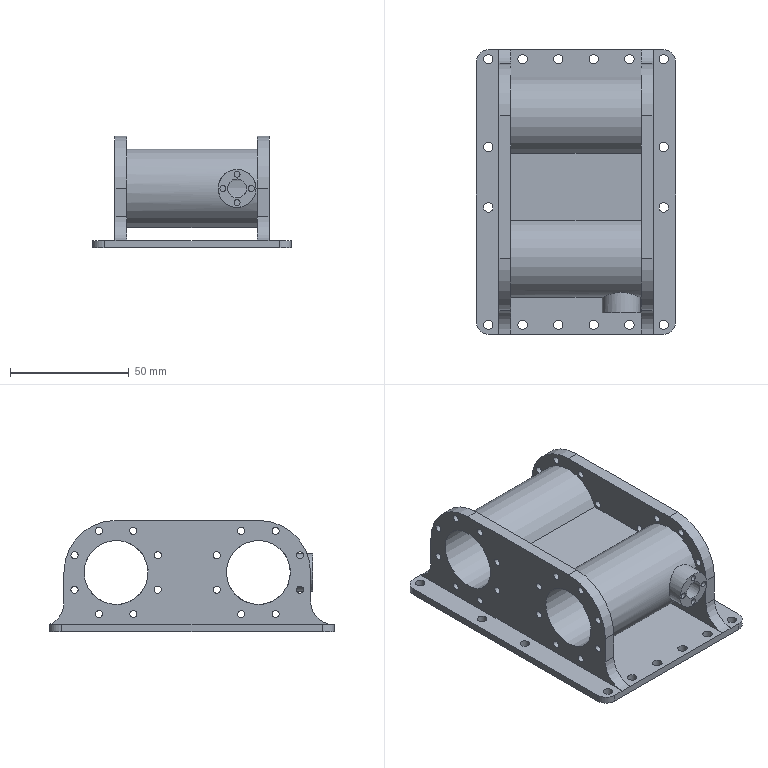Component | NX | PISTON_CYL_BODY | 1 solid | 95 faces | volume 108062 mm3 | cylinder 70 | plane 25 | commonest cylinder face diameters 3 x32 4 x16 44 x4 10 x4 20 x4 2.5 x4 33 x2 27 x2